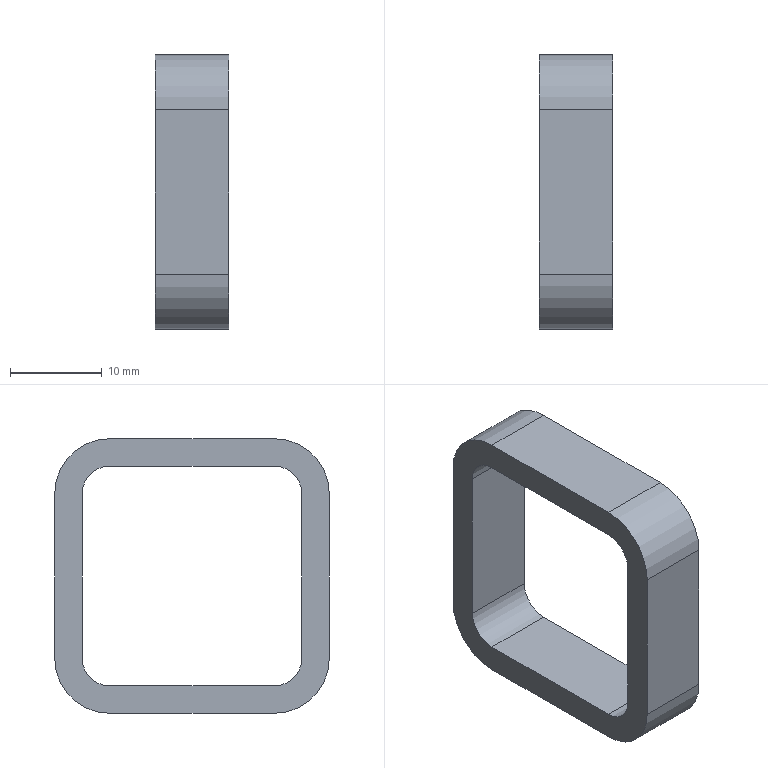Component | SolidWorks | MirrorRailing2-10_Mirror30X30X3-1100-3 | 1 solid | 18 faces | box 8 x 30 x 30 mm | volume 2407 mm3 | plane 10 | cylinder 8 | commonest cylinder face diameters 12 x4 6 x4
STEP:
#1=CARTESIAN_POINT('',(81.808,-890.067,3.898));
#2=VERTEX_POINT('',#1);
#3=CARTESIAN_POINT('',(81.808,-889.831,4.134));
#4=VERTEX_POINT('',#3);
#5=CARTESIAN_POINT('',(81.808,-890.067,4.134));
#6=DIRECTION('',(1.,0.,0.));
#7=DIRECTION('',(0.,0.,1.));
#8=AXIS2_PLACEMENT_3D('',#5,#6,#7);
#9=CIRCLE('',#8,0.2362);
#10=EDGE_CURVE('',#2,#4,#9,.T.);
#11=ORIENTED_EDGE('',*,*,#10,.F.);
#12=CARTESIAN_POINT('',(81.493,-890.067,3.898));
#13=VERTEX_POINT('',#12);
#14=CARTESIAN_POINT('',(124.8,-890.067,3.898));
#15=DIRECTION('',(-1.,0.,0.));
#16=VECTOR('',#15,39.37);
#17=LINE('',#14,#16);
#18=EDGE_CURVE('',#2,#13,#17,.T.);
#19=ORIENTED_EDGE('',*,*,#18,.T.);
#20=CARTESIAN_POINT('',(81.493,-889.831,4.134));
#21=VERTEX_POINT('',#20);
#22=CARTESIAN_POINT('',(81.493,-890.067,4.134));
#23=DIRECTION('',(-1.,0.,0.));
#24=DIRECTION('',(0.,0.,-1.));
#25=AXIS2_PLACEMENT_3D('',#22,#23,#24);
#26=CIRCLE('',#25,0.2362);
#27=EDGE_CURVE('',#21,#13,#26,.T.);
#28=ORIENTED_EDGE('',*,*,#27,.F.);
#29=CARTESIAN_POINT('',(124.8,-889.831,4.134));
#30=DIRECTION('',(-1.,0.,0.));
#31=VECTOR('',#30,39.37);
#32=LINE('',#29,#31);
#33=EDGE_CURVE('',#4,#21,#32,.T.);
#34=ORIENTED_EDGE('',*,*,#33,.F.);
#35=EDGE_LOOP('',(#11,#19,#28,#34));
#36=FACE_OUTER_BOUND('',#35,.T.);
#37=CARTESIAN_POINT('',(124.8,-890.067,4.134));
#38=DIRECTION('',(-1.,0.,0.));
#39=DIRECTION('',(0.,0.,1.));
#40=AXIS2_PLACEMENT_3D('',#37,#38,#39);
#41=CYLINDRICAL_SURFACE('',#40,0.2362);
#42=ADVANCED_FACE('',(#36),#41,.T.);
#43=CARTESIAN_POINT('',(81.808,-890.776,3.898));
#44=VERTEX_POINT('',#43);
#45=CARTESIAN_POINT('',(81.808,-890.067,3.898));
#46=DIRECTION('',(0.,1.,0.));
#47=VECTOR('',#46,39.37);
#48=LINE('',#45,#47);
#49=EDGE_CURVE('',#44,#2,#48,.T.);
#50=ORIENTED_EDGE('',*,*,#49,.F.);
#51=CARTESIAN_POINT('',(81.493,-890.776,3.898));
#52=VERTEX_POINT('',#51);
#53=CARTESIAN_POINT('',(124.8,-890.776,3.898));
#54=DIRECTION('',(-1.,0.,0.));
#55=VECTOR('',#54,39.37);
#56=LINE('',#53,#55);
#57=EDGE_CURVE('',#44,#52,#56,.T.);
#58=ORIENTED_EDGE('',*,*,#57,.T.);
#59=CARTESIAN_POINT('',(81.493,-890.067,3.898));
#60=DIRECTION('',(0.,-1.,0.));
#61=VECTOR('',#60,39.37);
#62=LINE('',#59,#61);
#63=EDGE_CURVE('',#13,#52,#62,.T.);
#64=ORIENTED_EDGE('',*,*,#63,.F.);
#65=ORIENTED_EDGE('',*,*,#18,.F.);
#66=EDGE_LOOP('',(#50,#58,#64,#65));
#67=FACE_OUTER_BOUND('',#66,.T.);
#68=CARTESIAN_POINT('',(124.8,-890.067,3.898));
#69=DIRECTION('',(0.,0.,1.));
#70=DIRECTION('',(0.,1.,0.));
#71=AXIS2_PLACEMENT_3D('',#68,#69,#70);
#72=PLANE('',#71);
#73=ADVANCED_FACE('',(#67),#72,.F.);
#74=CARTESIAN_POINT('',(81.808,-891.012,4.134));
#75=VERTEX_POINT('',#74);
#76=CARTESIAN_POINT('',(81.808,-890.776,4.134));
#77=DIRECTION('',(1.,0.,0.));
#78=DIRECTION('',(0.,0.,1.));
#79=AXIS2_PLACEMENT_3D('',#76,#77,#78);
#80=CIRCLE('',#79,0.2362);
#81=EDGE_CURVE('',#75,#44,#80,.T.);
#82=ORIENTED_EDGE('',*,*,#81,.F.);
#83=CARTESIAN_POINT('',(81.493,-891.012,4.134));
#84=VERTEX_POINT('',#83);
#85=CARTESIAN_POINT('',(124.8,-891.012,4.134));
#86=DIRECTION('',(-1.,0.,0.));
#87=VECTOR('',#86,39.37);
#88=LINE('',#85,#87);
#89=EDGE_CURVE('',#75,#84,#88,.T.);
#90=ORIENTED_EDGE('',*,*,#89,.T.);
#91=CARTESIAN_POINT('',(81.493,-890.776,4.134));
#92=DIRECTION('',(-1.,0.,0.));
#93=DIRECTION('',(0.,0.,-1.));
#94=AXIS2_PLACEMENT_3D('',#91,#92,#93);
#95=CIRCLE('',#94,0.2362);
#96=EDGE_CURVE('',#52,#84,#95,.T.);
#97=ORIENTED_EDGE('',*,*,#96,.F.);
#98=ORIENTED_EDGE('',*,*,#57,.F.);
#99=EDGE_LOOP('',(#82,#90,#97,#98));
#100=FACE_OUTER_BOUND('',#99,.T.);
#101=CARTESIAN_POINT('',(124.8,-890.776,4.134));
#102=DIRECTION('',(-1.,0.,0.));
#103=DIRECTION('',(0.,0.,1.));
#104=AXIS2_PLACEMENT_3D('',#101,#102,#103);
#105=CYLINDRICAL_SURFACE('',#104,0.2362);
#106=ADVANCED_FACE('',(#100),#105,.T.);
#107=CARTESIAN_POINT('',(81.808,-891.012,4.843));
#108=VERTEX_POINT('',#107);
#109=CARTESIAN_POINT('',(81.808,-891.012,4.843));
#110=DIRECTION('',(0.,0.,-1.));
#111=VECTOR('',#110,39.37);
#112=LINE('',#109,#111);
#113=EDGE_CURVE('',#108,#75,#112,.T.);
#114=ORIENTED_EDGE('',*,*,#113,.F.);
#115=CARTESIAN_POINT('',(81.493,-891.012,4.843));
#116=VERTEX_POINT('',#115);
#117=CARTESIAN_POINT('',(124.8,-891.012,4.843));
#118=DIRECTION('',(-1.,0.,0.));
#119=VECTOR('',#118,39.37);
#120=LINE('',#117,#119);
#121=EDGE_CURVE('',#108,#116,#120,.T.);
#122=ORIENTED_EDGE('',*,*,#121,.T.);
#123=CARTESIAN_POINT('',(81.493,-891.012,4.843));
#124=DIRECTION('',(0.,0.,1.));
#125=VECTOR('',#124,39.37);
#126=LINE('',#123,#125);
#127=EDGE_CURVE('',#84,#116,#126,.T.);
#128=ORIENTED_EDGE('',*,*,#127,.F.);
#129=ORIENTED_EDGE('',*,*,#89,.F.);
#130=EDGE_LOOP('',(#114,#122,#128,#129));
#131=FACE_OUTER_BOUND('',#130,.T.);
#132=CARTESIAN_POINT('',(124.8,-891.012,4.843));
#133=DIRECTION('',(0.,1.,0.));
#134=DIRECTION('',(0.,0.,-1.));
#135=AXIS2_PLACEMENT_3D('',#132,#133,#134);
#136=PLANE('',#135);
#137=ADVANCED_FACE('',(#131),#136,.F.);
#138=CARTESIAN_POINT('',(81.808,-890.776,5.079));
#139=VERTEX_POINT('',#138);
#140=CARTESIAN_POINT('',(81.808,-890.776,4.843));
#141=DIRECTION('',(1.,0.,0.));
#142=DIRECTION('',(0.,0.,1.));
#143=AXIS2_PLACEMENT_3D('',#140,#141,#142);
#144=CIRCLE('',#143,0.2362);
#145=EDGE_CURVE('',#139,#108,#144,.T.);
#146=ORIENTED_EDGE('',*,*,#145,.F.);
#147=CARTESIAN_POINT('',(81.493,-890.776,5.079));
#148=VERTEX_POINT('',#147);
#149=CARTESIAN_POINT('',(124.8,-890.776,5.079));
#150=DIRECTION('',(-1.,0.,0.));
#151=VECTOR('',#150,39.37);
#152=LINE('',#149,#151);
#153=EDGE_CURVE('',#139,#148,#152,.T.);
#154=ORIENTED_EDGE('',*,*,#153,.T.);
#155=CARTESIAN_POINT('',(81.493,-890.776,4.843));
#156=DIRECTION('',(-1.,0.,0.));
#157=DIRECTION('',(0.,0.,-1.));
#158=AXIS2_PLACEMENT_3D('',#155,#156,#157);
#159=CIRCLE('',#158,0.2362);
#160=EDGE_CURVE('',#116,#148,#159,.T.);
#161=ORIENTED_EDGE('',*,*,#160,.F.);
#162=ORIENTED_EDGE('',*,*,#121,.F.);
#163=EDGE_LOOP('',(#146,#154,#161,#162));
#164=FACE_OUTER_BOUND('',#163,.T.);
#165=CARTESIAN_POINT('',(124.8,-890.776,4.843));
#166=DIRECTION('',(-1.,0.,0.));
#167=DIRECTION('',(0.,0.,1.));
#168=AXIS2_PLACEMENT_3D('',#165,#166,#167);
#169=CYLINDRICAL_SURFACE('',#168,0.2362);
#170=ADVANCED_FACE('',(#164),#169,.T.);
#171=CARTESIAN_POINT('',(81.808,-890.067,5.079));
#172=VERTEX_POINT('',#171);
#173=CARTESIAN_POINT('',(81.808,-890.776,5.079));
#174=DIRECTION('',(0.,-1.,0.));
#175=VECTOR('',#174,39.37);
#176=LINE('',#173,#175);
#177=EDGE_CURVE('',#172,#139,#176,.T.);
#178=ORIENTED_EDGE('',*,*,#177,.F.);
#179=CARTESIAN_POINT('',(81.493,-890.067,5.079));
#180=VERTEX_POINT('',#179);
#181=CARTESIAN_POINT('',(124.8,-890.067,5.079));
#182=DIRECTION('',(-1.,0.,0.));
#183=VECTOR('',#182,39.37);
#184=LINE('',#181,#183);
#185=EDGE_CURVE('',#172,#180,#184,.T.);
#186=ORIENTED_EDGE('',*,*,#185,.T.);
#187=CARTESIAN_POINT('',(81.493,-890.776,5.079));
#188=DIRECTION('',(0.,1.,0.));
#189=VECTOR('',#188,39.37);
#190=LINE('',#187,#189);
#191=EDGE_CURVE('',#148,#180,#190,.T.);
#192=ORIENTED_EDGE('',*,*,#191,.F.);
#193=ORIENTED_EDGE('',*,*,#153,.F.);
#194=EDGE_LOOP('',(#178,#186,#192,#193));
#195=FACE_OUTER_BOUND('',#194,.T.);
#196=CARTESIAN_POINT('',(124.8,-890.776,5.079));
#197=DIRECTION('',(0.,0.,-1.));
#198=DIRECTION('',(0.,-1.,0.));
#199=AXIS2_PLACEMENT_3D('',#196,#197,#198);
#200=PLANE('',#199);
#201=ADVANCED_FACE('',(#195),#200,.F.);
#202=CARTESIAN_POINT('',(81.808,-889.831,4.843));
#203=VERTEX_POINT('',#202);
#204=CARTESIAN_POINT('',(81.808,-890.067,4.843));
#205=DIRECTION('',(1.,0.,0.));
#206=DIRECTION('',(0.,0.,1.));
#207=AXIS2_PLACEMENT_3D('',#204,#205,#206);
#208=CIRCLE('',#207,0.2362);
#209=EDGE_CURVE('',#203,#172,#208,.T.);
#210=ORIENTED_EDGE('',*,*,#209,.F.);
#211=CARTESIAN_POINT('',(81.493,-889.831,4.843));
#212=VERTEX_POINT('',#211);
#213=CARTESIAN_POINT('',(124.8,-889.831,4.843));
#214=DIRECTION('',(-1.,0.,0.));
#215=VECTOR('',#214,39.37);
#216=LINE('',#213,#215);
#217=EDGE_CURVE('',#203,#212,#216,.T.);
#218=ORIENTED_EDGE('',*,*,#217,.T.);
#219=CARTESIAN_POINT('',(81.493,-890.067,4.843));
#220=DIRECTION('',(-1.,0.,0.));
#221=DIRECTION('',(0.,0.,-1.));
#222=AXIS2_PLACEMENT_3D('',#219,#220,#221);
#223=CIRCLE('',#222,0.2362);
#224=EDGE_CURVE('',#180,#212,#223,.T.);
#225=ORIENTED_EDGE('',*,*,#224,.F.);
#226=ORIENTED_EDGE('',*,*,#185,.F.);
#227=EDGE_LOOP('',(#210,#218,#225,#226));
#228=FACE_OUTER_BOUND('',#227,.T.);
#229=CARTESIAN_POINT('',(124.8,-890.067,4.843));
#230=DIRECTION('',(-1.,0.,0.));
#231=DIRECTION('',(0.,0.,1.));
#232=AXIS2_PLACEMENT_3D('',#229,#230,#231);
#233=CYLINDRICAL_SURFACE('',#232,0.2362);
#234=ADVANCED_FACE('',(#228),#233,.T.);
#235=CARTESIAN_POINT('',(81.808,-890.894,4.134));
#236=VERTEX_POINT('',#235);
#237=CARTESIAN_POINT('',(81.493,-890.894,4.134));
#238=VERTEX_POINT('',#237);
#239=CARTESIAN_POINT('',(124.8,-890.894,4.134));
#240=DIRECTION('',(-1.,0.,0.));
#241=VECTOR('',#240,39.37);
#242=LINE('',#239,#241);
#243=EDGE_CURVE('',#236,#238,#242,.T.);
#244=ORIENTED_EDGE('',*,*,#243,.F.);
#245=CARTESIAN_POINT('',(81.808,-890.776,4.016));
#246=VERTEX_POINT('',#245);
#247=CARTESIAN_POINT('',(81.808,-890.776,4.134));
#248=DIRECTION('',(1.,0.,0.));
#249=DIRECTION('',(0.,0.,1.));
#250=AXIS2_PLACEMENT_3D('',#247,#248,#249);
#251=CIRCLE('',#250,0.1181);
#252=EDGE_CURVE('',#236,#246,#251,.T.);
#253=ORIENTED_EDGE('',*,*,#252,.T.);
#254=CARTESIAN_POINT('',(81.493,-890.776,4.016));
#255=VERTEX_POINT('',#254);
#256=CARTESIAN_POINT('',(124.8,-890.776,4.016));
#257=DIRECTION('',(-1.,0.,0.));
#258=VECTOR('',#257,39.37);
#259=LINE('',#256,#258);
#260=EDGE_CURVE('',#246,#255,#259,.T.);
#261=ORIENTED_EDGE('',*,*,#260,.T.);
#262=CARTESIAN_POINT('',(81.493,-890.776,4.134));
#263=DIRECTION('',(-1.,0.,0.));
#264=DIRECTION('',(0.,0.,-1.));
#265=AXIS2_PLACEMENT_3D('',#262,#263,#264);
#266=CIRCLE('',#265,0.1181);
#267=EDGE_CURVE('',#255,#238,#266,.T.);
#268=ORIENTED_EDGE('',*,*,#267,.T.);
#269=EDGE_LOOP('',(#244,#253,#261,#268));
#270=FACE_OUTER_BOUND('',#269,.T.);
#271=CARTESIAN_POINT('',(124.8,-890.776,4.134));
#272=DIRECTION('',(-1.,0.,0.));
#273=DIRECTION('',(0.,0.,1.));
#274=AXIS2_PLACEMENT_3D('',#271,#272,#273);
#275=CYLINDRICAL_SURFACE('',#274,0.1181);
#276=ADVANCED_FACE('',(#270),#275,.F.);
#277=ORIENTED_EDGE('',*,*,#260,.F.);
#278=CARTESIAN_POINT('',(81.808,-890.067,4.016));
#279=VERTEX_POINT('',#278);
#280=CARTESIAN_POINT('',(81.808,-890.067,4.016));
#281=DIRECTION('',(0.,1.,0.));
#282=VECTOR('',#281,39.37);
#283=LINE('',#280,#282);
#284=EDGE_CURVE('',#246,#279,#283,.T.);
#285=ORIENTED_EDGE('',*,*,#284,.T.);
#286=CARTESIAN_POINT('',(81.493,-890.067,4.016));
#287=VERTEX_POINT('',#286);
#288=CARTESIAN_POINT('',(124.8,-890.067,4.016));
#289=DIRECTION('',(-1.,0.,0.));
#290=VECTOR('',#289,39.37);
#291=LINE('',#288,#290);
#292=EDGE_CURVE('',#279,#287,#291,.T.);
#293=ORIENTED_EDGE('',*,*,#292,.T.);
#294=CARTESIAN_POINT('',(81.493,-890.067,4.016));
#295=DIRECTION('',(0.,-1.,0.));
#296=VECTOR('',#295,39.37);
#297=LINE('',#294,#296);
#298=EDGE_CURVE('',#287,#255,#297,.T.);
#299=ORIENTED_EDGE('',*,*,#298,.T.);
#300=EDGE_LOOP('',(#277,#285,#293,#299));
#301=FACE_OUTER_BOUND('',#300,.T.);
#302=CARTESIAN_POINT('',(124.8,-890.067,4.016));
#303=DIRECTION('',(0.,0.,1.));
#304=DIRECTION('',(0.,1.,0.));
#305=AXIS2_PLACEMENT_3D('',#302,#303,#304);
#306=PLANE('',#305);
#307=ADVANCED_FACE('',(#301),#306,.T.);
#308=ORIENTED_EDGE('',*,*,#292,.F.);
#309=CARTESIAN_POINT('',(81.808,-889.949,4.134));
#310=VERTEX_POINT('',#309);
#311=CARTESIAN_POINT('',(81.808,-890.067,4.134));
#312=DIRECTION('',(1.,0.,0.));
#313=DIRECTION('',(0.,0.,1.));
#314=AXIS2_PLACEMENT_3D('',#311,#312,#313);
#315=CIRCLE('',#314,0.1181);
#316=EDGE_CURVE('',#279,#310,#315,.T.);
#317=ORIENTED_EDGE('',*,*,#316,.T.);
#318=CARTESIAN_POINT('',(81.493,-889.949,4.134));
#319=VERTEX_POINT('',#318);
#320=CARTESIAN_POINT('',(124.8,-889.949,4.134));
#321=DIRECTION('',(-1.,0.,0.));
#322=VECTOR('',#321,39.37);
#323=LINE('',#320,#322);
#324=EDGE_CURVE('',#310,#319,#323,.T.);
#325=ORIENTED_EDGE('',*,*,#324,.T.);
#326=CARTESIAN_POINT('',(81.493,-890.067,4.134));
#327=DIRECTION('',(-1.,0.,0.));
#328=DIRECTION('',(0.,0.,-1.));
#329=AXIS2_PLACEMENT_3D('',#326,#327,#328);
#330=CIRCLE('',#329,0.1181);
#331=EDGE_CURVE('',#319,#287,#330,.T.);
#332=ORIENTED_EDGE('',*,*,#331,.T.);
#333=EDGE_LOOP('',(#308,#317,#325,#332));
#334=FACE_OUTER_BOUND('',#333,.T.);
#335=CARTESIAN_POINT('',(124.8,-890.067,4.134));
#336=DIRECTION('',(-1.,0.,0.));
#337=DIRECTION('',(0.,0.,1.));
#338=AXIS2_PLACEMENT_3D('',#335,#336,#337);
#339=CYLINDRICAL_SURFACE('',#338,0.1181);
#340=ADVANCED_FACE('',(#334),#339,.F.);
#341=ORIENTED_EDGE('',*,*,#324,.F.);
#342=CARTESIAN_POINT('',(81.808,-889.949,4.843));
#343=VERTEX_POINT('',#342);
#344=CARTESIAN_POINT('',(81.808,-889.949,4.134));
#345=DIRECTION('',(0.,0.,1.));
#346=VECTOR('',#345,39.37);
#347=LINE('',#344,#346);
#348=EDGE_CURVE('',#310,#343,#347,.T.);
#349=ORIENTED_EDGE('',*,*,#348,.T.);
#350=CARTESIAN_POINT('',(81.493,-889.949,4.843));
#351=VERTEX_POINT('',#350);
#352=CARTESIAN_POINT('',(124.8,-889.949,4.843));
#353=DIRECTION('',(-1.,0.,0.));
#354=VECTOR('',#353,39.37);
#355=LINE('',#352,#354);
#356=EDGE_CURVE('',#343,#351,#355,.T.);
#357=ORIENTED_EDGE('',*,*,#356,.T.);
#358=CARTESIAN_POINT('',(81.493,-889.949,4.134));
#359=DIRECTION('',(0.,0.,-1.));
#360=VECTOR('',#359,39.37);
#361=LINE('',#358,#360);
#362=EDGE_CURVE('',#351,#319,#361,.T.);
#363=ORIENTED_EDGE('',*,*,#362,.T.);
#364=EDGE_LOOP('',(#341,#349,#357,#363));
#365=FACE_OUTER_BOUND('',#364,.T.);
#366=CARTESIAN_POINT('',(124.8,-889.949,4.134));
#367=DIRECTION('',(0.,-1.,0.));
#368=DIRECTION('',(0.,0.,1.));
#369=AXIS2_PLACEMENT_3D('',#366,#367,#368);
#370=PLANE('',#369);
#371=ADVANCED_FACE('',(#365),#370,.T.);
#372=ORIENTED_EDGE('',*,*,#356,.F.);
#373=CARTESIAN_POINT('',(81.808,-890.067,4.961));
#374=VERTEX_POINT('',#373);
#375=CARTESIAN_POINT('',(81.808,-890.067,4.843));
#376=DIRECTION('',(1.,0.,0.));
#377=DIRECTION('',(0.,0.,1.));
#378=AXIS2_PLACEMENT_3D('',#375,#376,#377);
#379=CIRCLE('',#378,0.1181);
#380=EDGE_CURVE('',#343,#374,#379,.T.);
#381=ORIENTED_EDGE('',*,*,#380,.T.);
#382=CARTESIAN_POINT('',(81.493,-890.067,4.961));
#383=VERTEX_POINT('',#382);
#384=CARTESIAN_POINT('',(124.8,-890.067,4.961));
#385=DIRECTION('',(-1.,0.,0.));
#386=VECTOR('',#385,39.37);
#387=LINE('',#384,#386);
#388=EDGE_CURVE('',#374,#383,#387,.T.);
#389=ORIENTED_EDGE('',*,*,#388,.T.);
#390=CARTESIAN_POINT('',(81.493,-890.067,4.843));
#391=DIRECTION('',(-1.,0.,0.));
#392=DIRECTION('',(0.,0.,-1.));
#393=AXIS2_PLACEMENT_3D('',#390,#391,#392);
#394=CIRCLE('',#393,0.1181);
#395=EDGE_CURVE('',#383,#351,#394,.T.);
#396=ORIENTED_EDGE('',*,*,#395,.T.);
#397=EDGE_LOOP('',(#372,#381,#389,#396));
#398=FACE_OUTER_BOUND('',#397,.T.);
#399=CARTESIAN_POINT('',(124.8,-890.067,4.843));
#400=DIRECTION('',(-1.,0.,0.));
#401=DIRECTION('',(0.,0.,1.));
#402=AXIS2_PLACEMENT_3D('',#399,#400,#401);
#403=CYLINDRICAL_SURFACE('',#402,0.1181);
#404=ADVANCED_FACE('',(#398),#403,.F.);
#405=ORIENTED_EDGE('',*,*,#388,.F.);
#406=CARTESIAN_POINT('',(81.808,-890.776,4.961));
#407=VERTEX_POINT('',#406);
#408=CARTESIAN_POINT('',(81.808,-890.776,4.961));
#409=DIRECTION('',(0.,-1.,0.));
#410=VECTOR('',#409,39.37);
#411=LINE('',#408,#410);
#412=EDGE_CURVE('',#374,#407,#411,.T.);
#413=ORIENTED_EDGE('',*,*,#412,.T.);
#414=CARTESIAN_POINT('',(81.493,-890.776,4.961));
#415=VERTEX_POINT('',#414);
#416=CARTESIAN_POINT('',(124.8,-890.776,4.961));
#417=DIRECTION('',(-1.,0.,0.));
#418=VECTOR('',#417,39.37);
#419=LINE('',#416,#418);
#420=EDGE_CURVE('',#407,#415,#419,.T.);
#421=ORIENTED_EDGE('',*,*,#420,.T.);
#422=CARTESIAN_POINT('',(81.493,-890.776,4.961));
#423=DIRECTION('',(0.,1.,0.));
#424=VECTOR('',#423,39.37);
#425=LINE('',#422,#424);
#426=EDGE_CURVE('',#415,#383,#425,.T.);
#427=ORIENTED_EDGE('',*,*,#426,.T.);
#428=EDGE_LOOP('',(#405,#413,#421,#427));
#429=FACE_OUTER_BOUND('',#428,.T.);
#430=CARTESIAN_POINT('',(124.8,-890.776,4.961));
#431=DIRECTION('',(0.,0.,-1.));
#432=DIRECTION('',(0.,-1.,0.));
#433=AXIS2_PLACEMENT_3D('',#430,#431,#432);
#434=PLANE('',#433);
#435=ADVANCED_FACE('',(#429),#434,.T.);
#436=ORIENTED_EDGE('',*,*,#420,.F.);
#437=CARTESIAN_POINT('',(81.808,-890.894,4.843));
#438=VERTEX_POINT('',#437);
#439=CARTESIAN_POINT('',(81.808,-890.776,4.843));
#440=DIRECTION('',(1.,0.,0.));
#441=DIRECTION('',(0.,0.,1.));
#442=AXIS2_PLACEMENT_3D('',#439,#440,#441);
#443=CIRCLE('',#442,0.1181);
#444=EDGE_CURVE('',#407,#438,#443,.T.);
#445=ORIENTED_EDGE('',*,*,#444,.T.);
#446=CARTESIAN_POINT('',(81.493,-890.894,4.843));
#447=VERTEX_POINT('',#446);
#448=CARTESIAN_POINT('',(124.8,-890.894,4.843));
#449=DIRECTION('',(-1.,0.,0.));
#450=VECTOR('',#449,39.37);
#451=LINE('',#448,#450);
#452=EDGE_CURVE('',#438,#447,#451,.T.);
#453=ORIENTED_EDGE('',*,*,#452,.T.);
#454=CARTESIAN_POINT('',(81.493,-890.776,4.843));
#455=DIRECTION('',(-1.,0.,0.));
#456=DIRECTION('',(0.,0.,-1.));
#457=AXIS2_PLACEMENT_3D('',#454,#455,#456);
#458=CIRCLE('',#457,0.1181);
#459=EDGE_CURVE('',#447,#415,#458,.T.);
#460=ORIENTED_EDGE('',*,*,#459,.T.);
#461=EDGE_LOOP('',(#436,#445,#453,#460));
#462=FACE_OUTER_BOUND('',#461,.T.);
#463=CARTESIAN_POINT('',(124.8,-890.776,4.843));
#464=DIRECTION('',(-1.,0.,0.));
#465=DIRECTION('',(0.,0.,1.));
#466=AXIS2_PLACEMENT_3D('',#463,#464,#465);
#467=CYLINDRICAL_SURFACE('',#466,0.1181);
#468=ADVANCED_FACE('',(#462),#467,.F.);
#469=ORIENTED_EDGE('',*,*,#452,.F.);
#470=CARTESIAN_POINT('',(81.808,-890.894,4.843));
#471=DIRECTION('',(0.,0.,-1.));
#472=VECTOR('',#471,39.37);
#473=LINE('',#470,#472);
#474=EDGE_CURVE('',#438,#236,#473,.T.);
#475=ORIENTED_EDGE('',*,*,#474,.T.);
#476=ORIENTED_EDGE('',*,*,#243,.T.);
#477=CARTESIAN_POINT('',(81.493,-890.894,4.843));
#478=DIRECTION('',(0.,0.,1.));
#479=VECTOR('',#478,39.37);
#480=LINE('',#477,#479);
#481=EDGE_CURVE('',#238,#447,#480,.T.);
#482=ORIENTED_EDGE('',*,*,#481,.T.);
#483=EDGE_LOOP('',(#469,#475,#476,#482));
#484=FACE_OUTER_BOUND('',#483,.T.);
#485=CARTESIAN_POINT('',(124.8,-890.894,4.843));
#486=DIRECTION('',(0.,1.,0.));
#487=DIRECTION('',(0.,0.,-1.));
#488=AXIS2_PLACEMENT_3D('',#485,#486,#487);
#489=PLANE('',#488);
#490=ADVANCED_FACE('',(#484),#489,.T.);
#491=CARTESIAN_POINT('',(81.808,-889.831,4.134));
#492=DIRECTION('',(0.,0.,1.));
#493=VECTOR('',#492,39.37);
#494=LINE('',#491,#493);
#495=EDGE_CURVE('',#4,#203,#494,.T.);
#496=ORIENTED_EDGE('',*,*,#495,.F.);
#497=ORIENTED_EDGE('',*,*,#33,.T.);
#498=CARTESIAN_POINT('',(81.493,-889.831,4.134));
#499=DIRECTION('',(0.,0.,-1.));
#500=VECTOR('',#499,39.37);
#501=LINE('',#498,#500);
#502=EDGE_CURVE('',#212,#21,#501,.T.);
#503=ORIENTED_EDGE('',*,*,#502,.F.);
#504=ORIENTED_EDGE('',*,*,#217,.F.);
#505=EDGE_LOOP('',(#496,#497,#503,#504));
#506=FACE_OUTER_BOUND('',#505,.T.);
#507=CARTESIAN_POINT('',(124.8,-889.831,4.134));
#508=DIRECTION('',(0.,-1.,0.));
#509=DIRECTION('',(0.,0.,1.));
#510=AXIS2_PLACEMENT_3D('',#507,#508,#509);
#511=PLANE('',#510);
#512=ADVANCED_FACE('',(#506),#511,.F.);
#513=ORIENTED_EDGE('',*,*,#267,.F.);
#514=ORIENTED_EDGE('',*,*,#298,.F.);
#515=ORIENTED_EDGE('',*,*,#331,.F.);
#516=ORIENTED_EDGE('',*,*,#362,.F.);
#517=ORIENTED_EDGE('',*,*,#395,.F.);
#518=ORIENTED_EDGE('',*,*,#426,.F.);
#519=ORIENTED_EDGE('',*,*,#459,.F.);
#520=ORIENTED_EDGE('',*,*,#481,.F.);
#521=EDGE_LOOP('',(#513,#514,#515,#516,#517,#518,#519,#520));
#522=FACE_BOUND('',#521,.T.);
#523=ORIENTED_EDGE('',*,*,#27,.T.);
#524=ORIENTED_EDGE('',*,*,#63,.T.);
#525=ORIENTED_EDGE('',*,*,#96,.T.);
#526=ORIENTED_EDGE('',*,*,#127,.T.);
#527=ORIENTED_EDGE('',*,*,#160,.T.);
#528=ORIENTED_EDGE('',*,*,#191,.T.);
#529=ORIENTED_EDGE('',*,*,#224,.T.);
#530=ORIENTED_EDGE('',*,*,#502,.T.);
#531=EDGE_LOOP('',(#523,#524,#525,#526,#527,#528,#529,#530));
#532=FACE_OUTER_BOUND('',#531,.T.);
#533=CARTESIAN_POINT('',(81.493,-890.067,4.134));
#534=DIRECTION('',(1.,0.,0.));
#535=DIRECTION('',(0.,0.,-1.));
#536=AXIS2_PLACEMENT_3D('',#533,#534,#535);
#537=PLANE('',#536);
#538=ADVANCED_FACE('',(#522,#532),#537,.F.);
#539=ORIENTED_EDGE('',*,*,#474,.F.);
#540=ORIENTED_EDGE('',*,*,#444,.F.);
#541=ORIENTED_EDGE('',*,*,#412,.F.);
#542=ORIENTED_EDGE('',*,*,#380,.F.);
#543=ORIENTED_EDGE('',*,*,#348,.F.);
#544=ORIENTED_EDGE('',*,*,#316,.F.);
#545=ORIENTED_EDGE('',*,*,#284,.F.);
#546=ORIENTED_EDGE('',*,*,#252,.F.);
#547=EDGE_LOOP('',(#539,#540,#541,#542,#543,#544,#545,#546));
#548=FACE_BOUND('',#547,.T.);
#549=ORIENTED_EDGE('',*,*,#10,.T.);
#550=ORIENTED_EDGE('',*,*,#495,.T.);
#551=ORIENTED_EDGE('',*,*,#209,.T.);
#552=ORIENTED_EDGE('',*,*,#177,.T.);
#553=ORIENTED_EDGE('',*,*,#145,.T.);
#554=ORIENTED_EDGE('',*,*,#113,.T.);
#555=ORIENTED_EDGE('',*,*,#81,.T.);
#556=ORIENTED_EDGE('',*,*,#49,.T.);
#557=EDGE_LOOP('',(#549,#550,#551,#552,#553,#554,#555,#556));
#558=FACE_OUTER_BOUND('',#557,.T.);
#559=CARTESIAN_POINT('',(81.808,-862.094,5.607));
#560=DIRECTION('',(1.,0.,0.));
#561=DIRECTION('',(0.,0.,-1.));
#562=AXIS2_PLACEMENT_3D('',#559,#560,#561);
#563=PLANE('',#562);
#564=ADVANCED_FACE('',(#548,#558),#563,.T.);
#565=CLOSED_SHELL('',(#42,#73,#106,#137,#170,#201,#234,#276,#307,#340,#371,#404,#435,#468,#490,#512,#538,#564));
#566=MANIFOLD_SOLID_BREP('',#565);
#567=CARTESIAN_POINT('',(0.,0.,0.));
#568=DIRECTION('',(0.,0.,1.));
#569=DIRECTION('',(1.,0.,0.));
#570=AXIS2_PLACEMENT_3D('',#567,#568,#569);
#571=(LENGTH_UNIT()NAMED_UNIT(*)SI_UNIT($,.METRE.));
#572=LENGTH_MEASURE_WITH_UNIT(LENGTH_MEASURE(0.0254),#571);
#573=DIMENSIONAL_EXPONENTS(1.,0.,0.,0.,0.,0.,0.);
#574=(CONVERSION_BASED_UNIT('',#572)LENGTH_UNIT()NAMED_UNIT(#573));
#575=UNCERTAINTY_MEASURE_WITH_UNIT(LENGTH_MEASURE(0.00001),#574,'','');
#576=(NAMED_UNIT(*)PLANE_ANGLE_UNIT()SI_UNIT($,.RADIAN.));
#577=(NAMED_UNIT(*)SI_UNIT($,.STERADIAN.)SOLID_ANGLE_UNIT());
#578=(GEOMETRIC_REPRESENTATION_CONTEXT(3)GLOBAL_UNCERTAINTY_ASSIGNED_CONTEXT((#575))GLOBAL_UNIT_ASSIGNED_CONTEXT((#574,#576,#577))REPRESENTATION_CONTEXT('',''));
#579=ADVANCED_BREP_SHAPE_REPRESENTATION('',(#566,#570),#578);
#580=COLOUR_RGB('',0.7922,0.8196,0.9333);
#581=FILL_AREA_STYLE_COLOUR('',#580);
#582=FILL_AREA_STYLE('',(#581));
#583=SURFACE_STYLE_FILL_AREA(#582);
#584=SURFACE_SIDE_STYLE('',(#583));
#585=SURFACE_STYLE_USAGE(.BOTH.,#584);
#586=PRESENTATION_STYLE_ASSIGNMENT((#585));
#587=STYLED_ITEM('',(#586),#566);
#588=PRESENTATION_LAYER_ASSIGNMENT('','',(#587));
#589=(LENGTH_UNIT()NAMED_UNIT(*)SI_UNIT($,.METRE.));
#590=LENGTH_MEASURE_WITH_UNIT(LENGTH_MEASURE(0.0254),#589);
#591=DIMENSIONAL_EXPONENTS(1.,0.,0.,0.,0.,0.,0.);
#592=(CONVERSION_BASED_UNIT('',#590)LENGTH_UNIT()NAMED_UNIT(#591));
#593=UNCERTAINTY_MEASURE_WITH_UNIT(LENGTH_MEASURE(0.00001),#592,'','');
#594=(NAMED_UNIT(*)PLANE_ANGLE_UNIT()SI_UNIT($,.RADIAN.));
#595=(NAMED_UNIT(*)SI_UNIT($,.STERADIAN.)SOLID_ANGLE_UNIT());
#596=(GEOMETRIC_REPRESENTATION_CONTEXT(3)GLOBAL_UNCERTAINTY_ASSIGNED_CONTEXT((#593))GLOBAL_UNIT_ASSIGNED_CONTEXT((#592,#594,#595))REPRESENTATION_CONTEXT('',''));
#597=MECHANICAL_DESIGN_GEOMETRIC_PRESENTATION_REPRESENTATION('',(#587),#596);